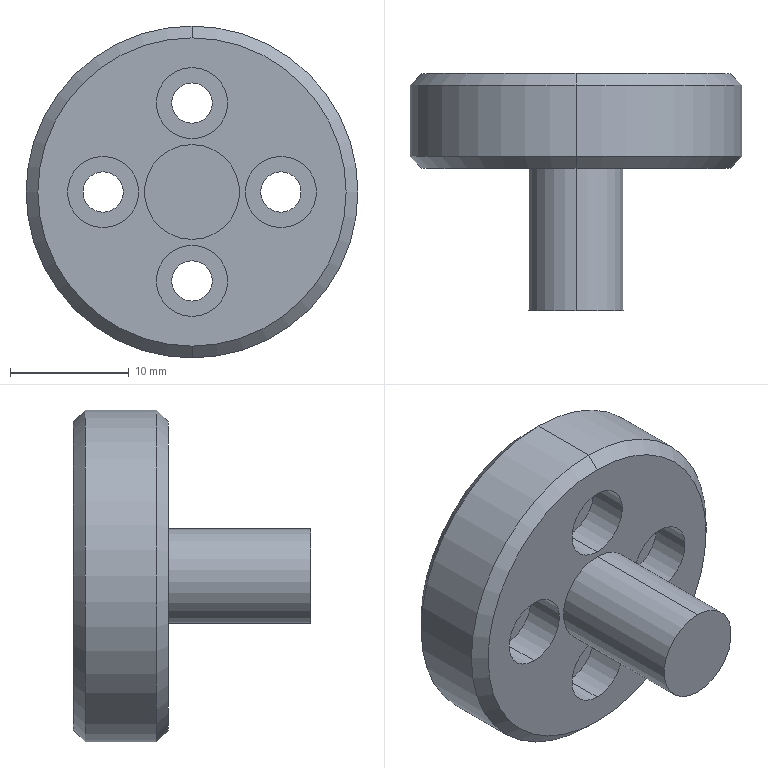Component | SolidWorks | H2020022-0438-1-1 | 1 solid | 34 faces | box 28 x 20 x 28 mm | volume 4336 mm3 | cylinder 22 | plane 8 | cone 4 | commonest cylinder face diameters 6 x8 3.4 x8 8 x2 20 x2 28 x2 | material 45#Steel
build123d program:
from build123d import *

# Parameters (mm, degrees)
SKETCH1_R                                       = 14
BOSS_EXTRUDE1_DEPTH                             = 8
SKETCH2_R                                       = 10
CUT_EXTRUDE1_DEPTH                              = 2
M3_HEX_SOCKET_HEAD_CAP_SCREW_CBORE1_D           = 3.4
M3_HEX_SOCKET_HEAD_CAP_SCREW_CBORE1_CBORE_D     = 6
M3_HEX_SOCKET_HEAD_CAP_SCREW_CBORE1_CBORE_DEPTH = 3.4
SKETCH5_R                                       = 4
BOSS_EXTRUDE2_DEPTH                             = 12
CHAMFER1_SIZE                                   = 1


with BuildPart() as part:
    # Sketch1 → Boss-Extrude1 (new body)
    with BuildSketch(Plane(origin=(0, 0, 0), x_dir=(1, 0, 0), z_dir=(0, 1, 0))):
        with Locations(Location((0, 0, 0), (0, 0, 270))):
            Circle(SKETCH1_R)
    extrude(amount=BOSS_EXTRUDE1_DEPTH)

    # Sketch2 → Cut-Extrude1 (cut)
    with BuildSketch(Plane(origin=(0, 8, 0), x_dir=(1, 0, 0), z_dir=(0, 1, 0))):
        with Locations(Location((0, 0, 0), (0, 0, 270))):
            Circle(SKETCH2_R)
    extrude(amount=-CUT_EXTRUDE1_DEPTH, mode=Mode.SUBTRACT)

    # M3 Hex Socket Head Cap Screw CBORE1 (through all)
    with Locations(Plane(origin=(0, 0, 0), x_dir=(-1, 0, 0), z_dir=(0, -1, 0))):
        with Locations((0, 7.5), (0, -7.5), (-7.5, 0), (7.5, 0)):
            CounterBoreHole(M3_HEX_SOCKET_HEAD_CAP_SCREW_CBORE1_D / 2, M3_HEX_SOCKET_HEAD_CAP_SCREW_CBORE1_CBORE_D / 2, M3_HEX_SOCKET_HEAD_CAP_SCREW_CBORE1_CBORE_DEPTH)

    # Sketch5 → Boss-Extrude2 (add)
    with BuildSketch(Plane.XZ):
        with Locations(Location((0, 0, 0), (0, 0, 90))):
            Circle(SKETCH5_R)
    extrude(amount=BOSS_EXTRUDE2_DEPTH)

    # Chamfer1
    chamfer1_edges = [part.edges().sort_by_distance(p)[0] for p in [
        (0, 0, -14),
        (0, 8, -14),
    ]]
    chamfer(chamfer1_edges, length=CHAMFER1_SIZE)


solid = part.part

# Placed as in the assembly
solid = solid.moved(Location((-30.964, 93.813, 280.197), (0, 0, 0)))
STEP:
#1=CARTESIAN_POINT('',(-1.219,4.008,11.543));
#2=VERTEX_POINT('',#1);
#3=CARTESIAN_POINT('',(-1.219,4.008,10.52));
#4=VERTEX_POINT('',#3);
#5=CARTESIAN_POINT('',(-1.219,4.008,11.031));
#6=DIRECTION('',(0.,1.,0.));
#7=DIRECTION('',(0.,0.,1.));
#8=AXIS2_PLACEMENT_3D('',#5,#6,#7);
#9=CIRCLE('',#8,0.5118);
#10=EDGE_CURVE('',#2,#4,#9,.T.);
#11=ORIENTED_EDGE('',*,*,#10,.F.);
#12=CARTESIAN_POINT('',(-1.219,3.969,11.583));
#13=VERTEX_POINT('',#12);
#14=CARTESIAN_POINT('',(-1.219,4.008,11.543));
#15=DIRECTION('',(0.,-0.7071,0.7071));
#16=VECTOR('',#15,39.37);
#17=LINE('',#14,#16);
#18=EDGE_CURVE('',#2,#13,#17,.T.);
#19=ORIENTED_EDGE('',*,*,#18,.T.);
#20=CARTESIAN_POINT('',(-1.219,3.969,10.48));
#21=VERTEX_POINT('',#20);
#22=CARTESIAN_POINT('',(-1.219,3.969,11.031));
#23=DIRECTION('',(0.,-1.,0.));
#24=DIRECTION('',(0.,0.,1.));
#25=AXIS2_PLACEMENT_3D('',#22,#23,#24);
#26=CIRCLE('',#25,0.5512);
#27=EDGE_CURVE('',#21,#13,#26,.T.);
#28=ORIENTED_EDGE('',*,*,#27,.F.);
#29=CARTESIAN_POINT('',(-1.219,4.008,10.52));
#30=DIRECTION('',(0.,-0.7071,-0.7071));
#31=VECTOR('',#30,39.37);
#32=LINE('',#29,#31);
#33=EDGE_CURVE('',#4,#21,#32,.T.);
#34=ORIENTED_EDGE('',*,*,#33,.F.);
#35=EDGE_LOOP('',(#11,#19,#28,#34));
#36=FACE_OUTER_BOUND('',#35,.T.);
#37=CARTESIAN_POINT('',(-1.219,4.008,11.031));
#38=DIRECTION('',(0.,-1.,0.));
#39=DIRECTION('',(0.,0.,-1.));
#40=AXIS2_PLACEMENT_3D('',#37,#38,#39);
#41=CONICAL_SURFACE('',#40,0.5118,0.7854);
#42=ADVANCED_FACE('',(#36),#41,.T.);
#43=CARTESIAN_POINT('',(-1.219,3.693,10.52));
#44=VERTEX_POINT('',#43);
#45=CARTESIAN_POINT('',(-1.219,3.693,11.543));
#46=VERTEX_POINT('',#45);
#47=CARTESIAN_POINT('',(-1.219,3.693,11.031));
#48=DIRECTION('',(0.,-1.,0.));
#49=DIRECTION('',(0.,0.,1.));
#50=AXIS2_PLACEMENT_3D('',#47,#48,#49);
#51=CIRCLE('',#50,0.5118);
#52=EDGE_CURVE('',#44,#46,#51,.T.);
#53=ORIENTED_EDGE('',*,*,#52,.F.);
#54=CARTESIAN_POINT('',(-1.219,3.733,10.48));
#55=VERTEX_POINT('',#54);
#56=CARTESIAN_POINT('',(-1.219,3.733,10.48));
#57=DIRECTION('',(0.,0.7071,-0.7071));
#58=VECTOR('',#57,39.37);
#59=LINE('',#56,#58);
#60=EDGE_CURVE('',#44,#55,#59,.T.);
#61=ORIENTED_EDGE('',*,*,#60,.T.);
#62=CARTESIAN_POINT('',(-1.219,3.733,11.583));
#63=VERTEX_POINT('',#62);
#64=CARTESIAN_POINT('',(-1.219,3.733,11.031));
#65=DIRECTION('',(0.,1.,0.));
#66=DIRECTION('',(0.,0.,1.));
#67=AXIS2_PLACEMENT_3D('',#64,#65,#66);
#68=CIRCLE('',#67,0.5512);
#69=EDGE_CURVE('',#63,#55,#68,.T.);
#70=ORIENTED_EDGE('',*,*,#69,.F.);
#71=CARTESIAN_POINT('',(-1.219,3.733,11.583));
#72=DIRECTION('',(0.,0.7071,0.7071));
#73=VECTOR('',#72,39.37);
#74=LINE('',#71,#73);
#75=EDGE_CURVE('',#46,#63,#74,.T.);
#76=ORIENTED_EDGE('',*,*,#75,.F.);
#77=EDGE_LOOP('',(#53,#61,#70,#76));
#78=FACE_OUTER_BOUND('',#77,.T.);
#79=CARTESIAN_POINT('',(-1.219,3.733,11.031));
#80=DIRECTION('',(0.,1.,0.));
#81=DIRECTION('',(0.,0.,1.));
#82=AXIS2_PLACEMENT_3D('',#79,#80,#81);
#83=CONICAL_SURFACE('',#82,0.5512,0.7854);
#84=ADVANCED_FACE('',(#78),#83,.T.);
#85=CARTESIAN_POINT('',(-1.219,3.221,10.874));
#86=VERTEX_POINT('',#85);
#87=CARTESIAN_POINT('',(-1.219,3.221,11.189));
#88=VERTEX_POINT('',#87);
#89=CARTESIAN_POINT('',(-1.219,3.221,11.031));
#90=DIRECTION('',(0.,-1.,0.));
#91=DIRECTION('',(0.,0.,-1.));
#92=AXIS2_PLACEMENT_3D('',#89,#90,#91);
#93=CIRCLE('',#92,0.1575);
#94=EDGE_CURVE('',#86,#88,#93,.T.);
#95=ORIENTED_EDGE('',*,*,#94,.F.);
#96=CARTESIAN_POINT('',(-1.219,3.693,10.874));
#97=VERTEX_POINT('',#96);
#98=CARTESIAN_POINT('',(-1.219,3.221,10.874));
#99=DIRECTION('',(0.,1.,0.));
#100=VECTOR('',#99,39.37);
#101=LINE('',#98,#100);
#102=EDGE_CURVE('',#86,#97,#101,.T.);
#103=ORIENTED_EDGE('',*,*,#102,.T.);
#104=CARTESIAN_POINT('',(-1.219,3.693,11.189));
#105=VERTEX_POINT('',#104);
#106=CARTESIAN_POINT('',(-1.219,3.693,11.031));
#107=DIRECTION('',(0.,-1.,0.));
#108=DIRECTION('',(0.,0.,1.));
#109=AXIS2_PLACEMENT_3D('',#106,#107,#108);
#110=CIRCLE('',#109,0.1575);
#111=EDGE_CURVE('',#97,#105,#110,.T.);
#112=ORIENTED_EDGE('',*,*,#111,.T.);
#113=CARTESIAN_POINT('',(-1.219,3.221,11.189));
#114=DIRECTION('',(0.,1.,0.));
#115=VECTOR('',#114,39.37);
#116=LINE('',#113,#115);
#117=EDGE_CURVE('',#88,#105,#116,.T.);
#118=ORIENTED_EDGE('',*,*,#117,.F.);
#119=EDGE_LOOP('',(#95,#103,#112,#118));
#120=FACE_OUTER_BOUND('',#119,.T.);
#121=CARTESIAN_POINT('',(-1.219,3.221,11.031));
#122=DIRECTION('',(0.,1.,0.));
#123=DIRECTION('',(0.,0.,1.));
#124=AXIS2_PLACEMENT_3D('',#121,#122,#123);
#125=CYLINDRICAL_SURFACE('',#124,0.1575);
#126=ADVANCED_FACE('',(#120),#125,.T.);
#127=CARTESIAN_POINT('',(-1.219,3.827,10.854));
#128=VERTEX_POINT('',#127);
#129=CARTESIAN_POINT('',(-1.219,3.827,10.618));
#130=VERTEX_POINT('',#129);
#131=CARTESIAN_POINT('',(-1.219,3.827,10.736));
#132=DIRECTION('',(0.,-1.,0.));
#133=DIRECTION('',(0.,0.,-1.));
#134=AXIS2_PLACEMENT_3D('',#131,#132,#133);
#135=CIRCLE('',#134,0.1181);
#136=EDGE_CURVE('',#128,#130,#135,.T.);
#137=ORIENTED_EDGE('',*,*,#136,.F.);
#138=CARTESIAN_POINT('',(-1.219,3.693,10.854));
#139=VERTEX_POINT('',#138);
#140=CARTESIAN_POINT('',(-1.219,3.693,10.854));
#141=DIRECTION('',(0.,-1.,0.));
#142=VECTOR('',#141,39.37);
#143=LINE('',#140,#142);
#144=EDGE_CURVE('',#128,#139,#143,.T.);
#145=ORIENTED_EDGE('',*,*,#144,.T.);
#146=CARTESIAN_POINT('',(-1.219,3.693,10.618));
#147=VERTEX_POINT('',#146);
#148=CARTESIAN_POINT('',(-1.219,3.693,10.736));
#149=DIRECTION('',(0.,-1.,0.));
#150=DIRECTION('',(0.,0.,-1.));
#151=AXIS2_PLACEMENT_3D('',#148,#149,#150);
#152=CIRCLE('',#151,0.1181);
#153=EDGE_CURVE('',#139,#147,#152,.T.);
#154=ORIENTED_EDGE('',*,*,#153,.T.);
#155=CARTESIAN_POINT('',(-1.219,3.693,10.618));
#156=DIRECTION('',(0.,-1.,0.));
#157=VECTOR('',#156,39.37);
#158=LINE('',#155,#157);
#159=EDGE_CURVE('',#130,#147,#158,.T.);
#160=ORIENTED_EDGE('',*,*,#159,.F.);
#161=EDGE_LOOP('',(#137,#145,#154,#160));
#162=FACE_OUTER_BOUND('',#161,.T.);
#163=CARTESIAN_POINT('',(-1.219,3.693,10.736));
#164=DIRECTION('',(0.,-1.,0.));
#165=DIRECTION('',(0.,0.,-1.));
#166=AXIS2_PLACEMENT_3D('',#163,#164,#165);
#167=CYLINDRICAL_SURFACE('',#166,0.1181);
#168=ADVANCED_FACE('',(#162),#167,.F.);
#169=CARTESIAN_POINT('',(-1.219,3.93,10.669));
#170=VERTEX_POINT('',#169);
#171=CARTESIAN_POINT('',(-1.219,3.93,10.803));
#172=VERTEX_POINT('',#171);
#173=CARTESIAN_POINT('',(-1.219,3.93,10.736));
#174=DIRECTION('',(0.,1.,0.));
#175=DIRECTION('',(0.,0.,1.));
#176=AXIS2_PLACEMENT_3D('',#173,#174,#175);
#177=CIRCLE('',#176,0.06693);
#178=EDGE_CURVE('',#170,#172,#177,.T.);
#179=ORIENTED_EDGE('',*,*,#178,.T.);
#180=CARTESIAN_POINT('',(-1.219,3.827,10.803));
#181=VERTEX_POINT('',#180);
#182=CARTESIAN_POINT('',(-1.219,3.693,10.803));
#183=DIRECTION('',(0.,-1.,0.));
#184=VECTOR('',#183,39.37);
#185=LINE('',#182,#184);
#186=EDGE_CURVE('',#172,#181,#185,.T.);
#187=ORIENTED_EDGE('',*,*,#186,.T.);
#188=CARTESIAN_POINT('',(-1.219,3.827,10.669));
#189=VERTEX_POINT('',#188);
#190=CARTESIAN_POINT('',(-1.219,3.827,10.736));
#191=DIRECTION('',(0.,-1.,0.));
#192=DIRECTION('',(0.,0.,-1.));
#193=AXIS2_PLACEMENT_3D('',#190,#191,#192);
#194=CIRCLE('',#193,0.06693);
#195=EDGE_CURVE('',#181,#189,#194,.T.);
#196=ORIENTED_EDGE('',*,*,#195,.T.);
#197=CARTESIAN_POINT('',(-1.219,3.693,10.669));
#198=DIRECTION('',(0.,-1.,0.));
#199=VECTOR('',#198,39.37);
#200=LINE('',#197,#199);
#201=EDGE_CURVE('',#170,#189,#200,.T.);
#202=ORIENTED_EDGE('',*,*,#201,.F.);
#203=EDGE_LOOP('',(#179,#187,#196,#202));
#204=FACE_OUTER_BOUND('',#203,.T.);
#205=CARTESIAN_POINT('',(-1.219,3.693,10.736));
#206=DIRECTION('',(0.,-1.,0.));
#207=DIRECTION('',(0.,0.,-1.));
#208=AXIS2_PLACEMENT_3D('',#205,#206,#207);
#209=CYLINDRICAL_SURFACE('',#208,0.06693);
#210=ADVANCED_FACE('',(#204),#209,.F.);
#211=CARTESIAN_POINT('',(-1.219,3.827,11.445));
#212=VERTEX_POINT('',#211);
#213=CARTESIAN_POINT('',(-1.219,3.827,11.209));
#214=VERTEX_POINT('',#213);
#215=CARTESIAN_POINT('',(-1.219,3.827,11.327));
#216=DIRECTION('',(0.,-1.,0.));
#217=DIRECTION('',(0.,0.,-1.));
#218=AXIS2_PLACEMENT_3D('',#215,#216,#217);
#219=CIRCLE('',#218,0.1181);
#220=EDGE_CURVE('',#212,#214,#219,.T.);
#221=ORIENTED_EDGE('',*,*,#220,.F.);
#222=CARTESIAN_POINT('',(-1.219,3.693,11.445));
#223=VERTEX_POINT('',#222);
#224=CARTESIAN_POINT('',(-1.219,3.693,11.445));
#225=DIRECTION('',(0.,-1.,0.));
#226=VECTOR('',#225,39.37);
#227=LINE('',#224,#226);
#228=EDGE_CURVE('',#212,#223,#227,.T.);
#229=ORIENTED_EDGE('',*,*,#228,.T.);
#230=CARTESIAN_POINT('',(-1.219,3.693,11.209));
#231=VERTEX_POINT('',#230);
#232=CARTESIAN_POINT('',(-1.219,3.693,11.327));
#233=DIRECTION('',(0.,-1.,0.));
#234=DIRECTION('',(0.,0.,-1.));
#235=AXIS2_PLACEMENT_3D('',#232,#233,#234);
#236=CIRCLE('',#235,0.1181);
#237=EDGE_CURVE('',#223,#231,#236,.T.);
#238=ORIENTED_EDGE('',*,*,#237,.T.);
#239=CARTESIAN_POINT('',(-1.219,3.693,11.209));
#240=DIRECTION('',(0.,-1.,0.));
#241=VECTOR('',#240,39.37);
#242=LINE('',#239,#241);
#243=EDGE_CURVE('',#214,#231,#242,.T.);
#244=ORIENTED_EDGE('',*,*,#243,.F.);
#245=EDGE_LOOP('',(#221,#229,#238,#244));
#246=FACE_OUTER_BOUND('',#245,.T.);
#247=CARTESIAN_POINT('',(-1.219,3.693,11.327));
#248=DIRECTION('',(0.,-1.,0.));
#249=DIRECTION('',(0.,0.,-1.));
#250=AXIS2_PLACEMENT_3D('',#247,#248,#249);
#251=CYLINDRICAL_SURFACE('',#250,0.1181);
#252=ADVANCED_FACE('',(#246),#251,.F.);
#253=CARTESIAN_POINT('',(-1.219,3.93,11.26));
#254=VERTEX_POINT('',#253);
#255=CARTESIAN_POINT('',(-1.219,3.93,11.394));
#256=VERTEX_POINT('',#255);
#257=CARTESIAN_POINT('',(-1.219,3.93,11.327));
#258=DIRECTION('',(0.,1.,0.));
#259=DIRECTION('',(0.,0.,1.));
#260=AXIS2_PLACEMENT_3D('',#257,#258,#259);
#261=CIRCLE('',#260,0.06693);
#262=EDGE_CURVE('',#254,#256,#261,.T.);
#263=ORIENTED_EDGE('',*,*,#262,.T.);
#264=CARTESIAN_POINT('',(-1.219,3.827,11.394));
#265=VERTEX_POINT('',#264);
#266=CARTESIAN_POINT('',(-1.219,3.693,11.394));
#267=DIRECTION('',(0.,-1.,0.));
#268=VECTOR('',#267,39.37);
#269=LINE('',#266,#268);
#270=EDGE_CURVE('',#256,#265,#269,.T.);
#271=ORIENTED_EDGE('',*,*,#270,.T.);
#272=CARTESIAN_POINT('',(-1.219,3.827,11.26));
#273=VERTEX_POINT('',#272);
#274=CARTESIAN_POINT('',(-1.219,3.827,11.327));
#275=DIRECTION('',(0.,-1.,0.));
#276=DIRECTION('',(0.,0.,-1.));
#277=AXIS2_PLACEMENT_3D('',#274,#275,#276);
#278=CIRCLE('',#277,0.06693);
#279=EDGE_CURVE('',#265,#273,#278,.T.);
#280=ORIENTED_EDGE('',*,*,#279,.T.);
#281=CARTESIAN_POINT('',(-1.219,3.693,11.26));
#282=DIRECTION('',(0.,-1.,0.));
#283=VECTOR('',#282,39.37);
#284=LINE('',#281,#283);
#285=EDGE_CURVE('',#254,#273,#284,.T.);
#286=ORIENTED_EDGE('',*,*,#285,.F.);
#287=EDGE_LOOP('',(#263,#271,#280,#286));
#288=FACE_OUTER_BOUND('',#287,.T.);
#289=CARTESIAN_POINT('',(-1.219,3.693,11.327));
#290=DIRECTION('',(0.,-1.,0.));
#291=DIRECTION('',(0.,0.,-1.));
#292=AXIS2_PLACEMENT_3D('',#289,#290,#291);
#293=CYLINDRICAL_SURFACE('',#292,0.06693);
#294=ADVANCED_FACE('',(#288),#293,.F.);
#295=CARTESIAN_POINT('',(-0.9238,3.827,11.149));
#296=VERTEX_POINT('',#295);
#297=CARTESIAN_POINT('',(-0.9238,3.827,10.913));
#298=VERTEX_POINT('',#297);
#299=CARTESIAN_POINT('',(-0.9238,3.827,11.031));
#300=DIRECTION('',(0.,-1.,0.));
#301=DIRECTION('',(0.,0.,-1.));
#302=AXIS2_PLACEMENT_3D('',#299,#300,#301);
#303=CIRCLE('',#302,0.1181);
#304=EDGE_CURVE('',#296,#298,#303,.T.);
#305=ORIENTED_EDGE('',*,*,#304,.F.);
#306=CARTESIAN_POINT('',(-0.9238,3.693,11.149));
#307=VERTEX_POINT('',#306);
#308=CARTESIAN_POINT('',(-0.9238,3.693,11.149));
#309=DIRECTION('',(0.,-1.,0.));
#310=VECTOR('',#309,39.37);
#311=LINE('',#308,#310);
#312=EDGE_CURVE('',#296,#307,#311,.T.);
#313=ORIENTED_EDGE('',*,*,#312,.T.);
#314=CARTESIAN_POINT('',(-0.9238,3.693,10.913));
#315=VERTEX_POINT('',#314);
#316=CARTESIAN_POINT('',(-0.9238,3.693,11.031));
#317=DIRECTION('',(0.,-1.,0.));
#318=DIRECTION('',(0.,0.,-1.));
#319=AXIS2_PLACEMENT_3D('',#316,#317,#318);
#320=CIRCLE('',#319,0.1181);
#321=EDGE_CURVE('',#307,#315,#320,.T.);
#322=ORIENTED_EDGE('',*,*,#321,.T.);
#323=CARTESIAN_POINT('',(-0.9238,3.693,10.913));
#324=DIRECTION('',(0.,-1.,0.));
#325=VECTOR('',#324,39.37);
#326=LINE('',#323,#325);
#327=EDGE_CURVE('',#298,#315,#326,.T.);
#328=ORIENTED_EDGE('',*,*,#327,.F.);
#329=EDGE_LOOP('',(#305,#313,#322,#328));
#330=FACE_OUTER_BOUND('',#329,.T.);
#331=CARTESIAN_POINT('',(-0.9238,3.693,11.031));
#332=DIRECTION('',(0.,-1.,0.));
#333=DIRECTION('',(0.,0.,-1.));
#334=AXIS2_PLACEMENT_3D('',#331,#332,#333);
#335=CYLINDRICAL_SURFACE('',#334,0.1181);
#336=ADVANCED_FACE('',(#330),#335,.F.);
#337=CARTESIAN_POINT('',(-0.9238,3.93,10.964));
#338=VERTEX_POINT('',#337);
#339=CARTESIAN_POINT('',(-0.9238,3.93,11.098));
#340=VERTEX_POINT('',#339);
#341=CARTESIAN_POINT('',(-0.9238,3.93,11.031));
#342=DIRECTION('',(0.,1.,0.));
#343=DIRECTION('',(0.,0.,1.));
#344=AXIS2_PLACEMENT_3D('',#341,#342,#343);
#345=CIRCLE('',#344,0.06693);
#346=EDGE_CURVE('',#338,#340,#345,.T.);
#347=ORIENTED_EDGE('',*,*,#346,.T.);
#348=CARTESIAN_POINT('',(-0.9238,3.827,11.098));
#349=VERTEX_POINT('',#348);
#350=CARTESIAN_POINT('',(-0.9238,3.693,11.098));
#351=DIRECTION('',(0.,-1.,0.));
#352=VECTOR('',#351,39.37);
#353=LINE('',#350,#352);
#354=EDGE_CURVE('',#340,#349,#353,.T.);
#355=ORIENTED_EDGE('',*,*,#354,.T.);
#356=CARTESIAN_POINT('',(-0.9238,3.827,10.964));
#357=VERTEX_POINT('',#356);
#358=CARTESIAN_POINT('',(-0.9238,3.827,11.031));
#359=DIRECTION('',(0.,-1.,0.));
#360=DIRECTION('',(0.,0.,-1.));
#361=AXIS2_PLACEMENT_3D('',#358,#359,#360);
#362=CIRCLE('',#361,0.06693);
#363=EDGE_CURVE('',#349,#357,#362,.T.);
#364=ORIENTED_EDGE('',*,*,#363,.T.);
#365=CARTESIAN_POINT('',(-0.9238,3.693,10.964));
#366=DIRECTION('',(0.,-1.,0.));
#367=VECTOR('',#366,39.37);
#368=LINE('',#365,#367);
#369=EDGE_CURVE('',#338,#357,#368,.T.);
#370=ORIENTED_EDGE('',*,*,#369,.F.);
#371=EDGE_LOOP('',(#347,#355,#364,#370));
#372=FACE_OUTER_BOUND('',#371,.T.);
#373=CARTESIAN_POINT('',(-0.9238,3.693,11.031));
#374=DIRECTION('',(0.,-1.,0.));
#375=DIRECTION('',(0.,0.,-1.));
#376=AXIS2_PLACEMENT_3D('',#373,#374,#375);
#377=CYLINDRICAL_SURFACE('',#376,0.06693);
#378=ADVANCED_FACE('',(#372),#377,.F.);
#379=CARTESIAN_POINT('',(-1.514,3.827,11.149));
#380=VERTEX_POINT('',#379);
#381=CARTESIAN_POINT('',(-1.514,3.827,10.913));
#382=VERTEX_POINT('',#381);
#383=CARTESIAN_POINT('',(-1.514,3.827,11.031));
#384=DIRECTION('',(0.,-1.,0.));
#385=DIRECTION('',(0.,0.,-1.));
#386=AXIS2_PLACEMENT_3D('',#383,#384,#385);
#387=CIRCLE('',#386,0.1181);
#388=EDGE_CURVE('',#380,#382,#387,.T.);
#389=ORIENTED_EDGE('',*,*,#388,.F.);
#390=CARTESIAN_POINT('',(-1.514,3.693,11.149));
#391=VERTEX_POINT('',#390);
#392=CARTESIAN_POINT('',(-1.514,3.693,11.149));
#393=DIRECTION('',(0.,-1.,0.));
#394=VECTOR('',#393,39.37);
#395=LINE('',#392,#394);
#396=EDGE_CURVE('',#380,#391,#395,.T.);
#397=ORIENTED_EDGE('',*,*,#396,.T.);
#398=CARTESIAN_POINT('',(-1.514,3.693,10.913));
#399=VERTEX_POINT('',#398);
#400=CARTESIAN_POINT('',(-1.514,3.693,11.031));
#401=DIRECTION('',(0.,-1.,0.));
#402=DIRECTION('',(0.,0.,-1.));
#403=AXIS2_PLACEMENT_3D('',#400,#401,#402);
#404=CIRCLE('',#403,0.1181);
#405=EDGE_CURVE('',#391,#399,#404,.T.);
#406=ORIENTED_EDGE('',*,*,#405,.T.);
#407=CARTESIAN_POINT('',(-1.514,3.693,10.913));
#408=DIRECTION('',(0.,-1.,0.));
#409=VECTOR('',#408,39.37);
#410=LINE('',#407,#409);
#411=EDGE_CURVE('',#382,#399,#410,.T.);
#412=ORIENTED_EDGE('',*,*,#411,.F.);
#413=EDGE_LOOP('',(#389,#397,#406,#412));
#414=FACE_OUTER_BOUND('',#413,.T.);
#415=CARTESIAN_POINT('',(-1.514,3.693,11.031));
#416=DIRECTION('',(0.,-1.,0.));
#417=DIRECTION('',(0.,0.,-1.));
#418=AXIS2_PLACEMENT_3D('',#415,#416,#417);
#419=CYLINDRICAL_SURFACE('',#418,0.1181);
#420=ADVANCED_FACE('',(#414),#419,.F.);
#421=CARTESIAN_POINT('',(-1.514,3.93,10.964));
#422=VERTEX_POINT('',#421);
#423=CARTESIAN_POINT('',(-1.514,3.93,11.098));
#424=VERTEX_POINT('',#423);
#425=CARTESIAN_POINT('',(-1.514,3.93,11.031));
#426=DIRECTION('',(0.,1.,0.));
#427=DIRECTION('',(0.,0.,1.));
#428=AXIS2_PLACEMENT_3D('',#425,#426,#427);
#429=CIRCLE('',#428,0.06693);
#430=EDGE_CURVE('',#422,#424,#429,.T.);
#431=ORIENTED_EDGE('',*,*,#430,.T.);
#432=CARTESIAN_POINT('',(-1.514,3.827,11.098));
#433=VERTEX_POINT('',#432);
#434=CARTESIAN_POINT('',(-1.514,3.693,11.098));
#435=DIRECTION('',(0.,-1.,0.));
#436=VECTOR('',#435,39.37);
#437=LINE('',#434,#436);
#438=EDGE_CURVE('',#424,#433,#437,.T.);
#439=ORIENTED_EDGE('',*,*,#438,.T.);
#440=CARTESIAN_POINT('',(-1.514,3.827,10.964));
#441=VERTEX_POINT('',#440);
#442=CARTESIAN_POINT('',(-1.514,3.827,11.031));
#443=DIRECTION('',(0.,-1.,0.));
#444=DIRECTION('',(0.,0.,-1.));
#445=AXIS2_PLACEMENT_3D('',#442,#443,#444);
#446=CIRCLE('',#445,0.06693);
#447=EDGE_CURVE('',#433,#441,#446,.T.);
#448=ORIENTED_EDGE('',*,*,#447,.T.);
#449=CARTESIAN_POINT('',(-1.514,3.693,10.964));
#450=DIRECTION('',(0.,-1.,0.));
#451=VECTOR('',#450,39.37);
#452=LINE('',#449,#451);
#453=EDGE_CURVE('',#422,#441,#452,.T.);
#454=ORIENTED_EDGE('',*,*,#453,.F.);
#455=EDGE_LOOP('',(#431,#439,#448,#454));
#456=FACE_OUTER_BOUND('',#455,.T.);
#457=CARTESIAN_POINT('',(-1.514,3.693,11.031));
#458=DIRECTION('',(0.,-1.,0.));
#459=DIRECTION('',(0.,0.,-1.));
#460=AXIS2_PLACEMENT_3D('',#457,#458,#459);
#461=CYLINDRICAL_SURFACE('',#460,0.06693);
#462=ADVANCED_FACE('',(#456),#461,.F.);
#463=CARTESIAN_POINT('',(-1.219,3.93,10.638));
#464=VERTEX_POINT('',#463);
#465=CARTESIAN_POINT('',(-1.219,3.93,11.425));
#466=VERTEX_POINT('',#465);
#467=CARTESIAN_POINT('',(-1.219,3.93,11.031));
#468=DIRECTION('',(0.,1.,0.));
#469=DIRECTION('',(0.,0.,1.));
#470=AXIS2_PLACEMENT_3D('',#467,#468,#469);
#471=CIRCLE('',#470,0.3937);
#472=EDGE_CURVE('',#464,#466,#471,.T.);
#473=ORIENTED_EDGE('',*,*,#472,.F.);
#474=CARTESIAN_POINT('',(-1.219,4.008,10.638));
#475=VERTEX_POINT('',#474);
#476=CARTESIAN_POINT('',(-1.219,3.93,10.638));
#477=DIRECTION('',(0.,1.,0.));
#478=VECTOR('',#477,39.37);
#479=LINE('',#476,#478);
#480=EDGE_CURVE('',#464,#475,#479,.T.);
#481=ORIENTED_EDGE('',*,*,#480,.T.);
#482=CARTESIAN_POINT('',(-1.219,4.008,11.425));
#483=VERTEX_POINT('',#482);
#484=CARTESIAN_POINT('',(-1.219,4.008,11.031));
#485=DIRECTION('',(0.,1.,0.));
#486=DIRECTION('',(0.,0.,1.));
#487=AXIS2_PLACEMENT_3D('',#484,#485,#486);
#488=CIRCLE('',#487,0.3937);
#489=EDGE_CURVE('',#475,#483,#488,.T.);
#490=ORIENTED_EDGE('',*,*,#489,.T.);
#491=CARTESIAN_POINT('',(-1.219,3.93,11.425));
#492=DIRECTION('',(0.,1.,0.));
#493=VECTOR('',#492,39.37);
#494=LINE('',#491,#493);
#495=EDGE_CURVE('',#466,#483,#494,.T.);
#496=ORIENTED_EDGE('',*,*,#495,.F.);
#497=EDGE_LOOP('',(#473,#481,#490,#496));
#498=FACE_OUTER_BOUND('',#497,.T.);
#499=CARTESIAN_POINT('',(-1.219,3.93,11.031));
#500=DIRECTION('',(0.,1.,0.));
#501=DIRECTION('',(0.,0.,1.));
#502=AXIS2_PLACEMENT_3D('',#499,#500,#501);
#503=CYLINDRICAL_SURFACE('',#502,0.3937);
#504=ADVANCED_FACE('',(#498),#503,.F.);
#505=ORIENTED_EDGE('',*,*,#27,.T.);
#506=CARTESIAN_POINT('',(-1.219,4.008,11.583));
#507=DIRECTION('',(0.,-1.,0.));
#508=VECTOR('',#507,39.37);
#509=LINE('',#506,#508);
#510=EDGE_CURVE('',#13,#63,#509,.T.);
#511=ORIENTED_EDGE('',*,*,#510,.T.);
#512=ORIENTED_EDGE('',*,*,#69,.T.);
#513=CARTESIAN_POINT('',(-1.219,4.008,10.48));
#514=DIRECTION('',(0.,-1.,0.));
#515=VECTOR('',#514,39.37);
#516=LINE('',#513,#515);
#517=EDGE_CURVE('',#21,#55,#516,.T.);
#518=ORIENTED_EDGE('',*,*,#517,.F.);
#519=EDGE_LOOP('',(#505,#511,#512,#518));
#520=FACE_OUTER_BOUND('',#519,.T.);
#521=CARTESIAN_POINT('',(-1.219,4.008,11.031));
#522=DIRECTION('',(0.,-1.,0.));
#523=DIRECTION('',(0.,0.,-1.));
#524=AXIS2_PLACEMENT_3D('',#521,#522,#523);
#525=CYLINDRICAL_SURFACE('',#524,0.5512);
#526=ADVANCED_FACE('',(#520),#525,.T.);
#527=ORIENTED_EDGE('',*,*,#510,.F.);
#528=CARTESIAN_POINT('',(-1.219,3.969,11.031));
#529=DIRECTION('',(0.,-1.,0.));
#530=DIRECTION('',(0.,0.,1.));
#531=AXIS2_PLACEMENT_3D('',#528,#529,#530);
#532=CIRCLE('',#531,0.5512);
#533=EDGE_CURVE('',#13,#21,#532,.T.);
#534=ORIENTED_EDGE('',*,*,#533,.T.);
#535=ORIENTED_EDGE('',*,*,#517,.T.);
#536=CARTESIAN_POINT('',(-1.219,3.733,11.031));
#537=DIRECTION('',(0.,1.,0.));
#538=DIRECTION('',(0.,0.,1.));
#539=AXIS2_PLACEMENT_3D('',#536,#537,#538);
#540=CIRCLE('',#539,0.5512);
#541=EDGE_CURVE('',#55,#63,#540,.T.);
#542=ORIENTED_EDGE('',*,*,#541,.T.);
#543=EDGE_LOOP('',(#527,#534,#535,#542));
#544=FACE_OUTER_BOUND('',#543,.T.);
#545=CARTESIAN_POINT('',(-1.219,4.008,11.031));
#546=DIRECTION('',(0.,-1.,0.));
#547=DIRECTION('',(0.,0.,-1.));
#548=AXIS2_PLACEMENT_3D('',#545,#546,#547);
#549=CYLINDRICAL_SURFACE('',#548,0.5512);
#550=ADVANCED_FACE('',(#544),#549,.T.);
#551=CARTESIAN_POINT('',(-1.219,4.008,11.031));
#552=DIRECTION('',(0.,1.,0.));
#553=DIRECTION('',(0.,0.,1.));
#554=AXIS2_PLACEMENT_3D('',#551,#552,#553);
#555=CIRCLE('',#554,0.5118);
#556=EDGE_CURVE('',#4,#2,#555,.T.);
#557=ORIENTED_EDGE('',*,*,#556,.T.);
#558=ORIENTED_EDGE('',*,*,#10,.T.);
#559=EDGE_LOOP('',(#557,#558));
#560=FACE_OUTER_BOUND('',#559,.T.);
#561=CARTESIAN_POINT('',(-1.219,4.008,11.031));
#562=DIRECTION('',(0.,1.,0.));
#563=DIRECTION('',(0.,0.,1.));
#564=AXIS2_PLACEMENT_3D('',#561,#562,#563);
#565=CIRCLE('',#564,0.3937);
#566=EDGE_CURVE('',#483,#475,#565,.T.);
#567=ORIENTED_EDGE('',*,*,#566,.F.);
#568=ORIENTED_EDGE('',*,*,#489,.F.);
#569=EDGE_LOOP('',(#567,#568));
#570=FACE_BOUND('',#569,.T.);
#571=CARTESIAN_POINT('',(-1.219,4.008,11.031));
#572=DIRECTION('',(0.,1.,0.));
#573=DIRECTION('',(0.,0.,1.));
#574=AXIS2_PLACEMENT_3D('',#571,#572,#573);
#575=PLANE('',#574);
#576=ADVANCED_FACE('',(#560,#570),#575,.T.);
#577=CARTESIAN_POINT('',(-1.219,3.693,11.031));
#578=DIRECTION('',(0.,-1.,0.));
#579=DIRECTION('',(0.,0.,1.));
#580=AXIS2_PLACEMENT_3D('',#577,#578,#579);
#581=CIRCLE('',#580,0.5118);
#582=EDGE_CURVE('',#46,#44,#581,.T.);
#583=ORIENTED_EDGE('',*,*,#582,.T.);
#584=ORIENTED_EDGE('',*,*,#52,.T.);
#585=EDGE_LOOP('',(#583,#584));
#586=FACE_OUTER_BOUND('',#585,.T.);
#587=CARTESIAN_POINT('',(-1.219,3.693,11.031));
#588=DIRECTION('',(0.,-1.,0.));
#589=DIRECTION('',(0.,0.,1.));
#590=AXIS2_PLACEMENT_3D('',#587,#588,#589);
#591=CIRCLE('',#590,0.1575);
#592=EDGE_CURVE('',#105,#97,#591,.T.);
#593=ORIENTED_EDGE('',*,*,#592,.F.);
#594=ORIENTED_EDGE('',*,*,#111,.F.);
#595=EDGE_LOOP('',(#593,#594));
#596=FACE_BOUND('',#595,.T.);
#597=CARTESIAN_POINT('',(-1.219,3.693,10.736));
#598=DIRECTION('',(0.,-1.,0.));
#599=DIRECTION('',(0.,0.,-1.));
#600=AXIS2_PLACEMENT_3D('',#597,#598,#599);
#601=CIRCLE('',#600,0.1181);
#602=EDGE_CURVE('',#147,#139,#601,.T.);
#603=ORIENTED_EDGE('',*,*,#602,.F.);
#604=ORIENTED_EDGE('',*,*,#153,.F.);
#605=EDGE_LOOP('',(#603,#604));
#606=FACE_BOUND('',#605,.T.);
#607=CARTESIAN_POINT('',(-1.219,3.693,11.327));
#608=DIRECTION('',(0.,-1.,0.));
#609=DIRECTION('',(0.,0.,-1.));
#610=AXIS2_PLACEMENT_3D('',#607,#608,#609);
#611=CIRCLE('',#610,0.1181);
#612=EDGE_CURVE('',#231,#223,#611,.T.);
#613=ORIENTED_EDGE('',*,*,#612,.F.);
#614=ORIENTED_EDGE('',*,*,#237,.F.);
#615=EDGE_LOOP('',(#613,#614));
#616=FACE_BOUND('',#615,.T.);
#617=CARTESIAN_POINT('',(-0.9238,3.693,11.031));
#618=DIRECTION('',(0.,-1.,0.));
#619=DIRECTION('',(0.,0.,-1.));
#620=AXIS2_PLACEMENT_3D('',#617,#618,#619);
#621=CIRCLE('',#620,0.1181);
#622=EDGE_CURVE('',#315,#307,#621,.T.);
#623=ORIENTED_EDGE('',*,*,#622,.F.);
#624=ORIENTED_EDGE('',*,*,#321,.F.);
#625=EDGE_LOOP('',(#623,#624));
#626=FACE_BOUND('',#625,.T.);
#627=CARTESIAN_POINT('',(-1.514,3.693,11.031));
#628=DIRECTION('',(0.,-1.,0.));
#629=DIRECTION('',(0.,0.,-1.));
#630=AXIS2_PLACEMENT_3D('',#627,#628,#629);
#631=CIRCLE('',#630,0.1181);
#632=EDGE_CURVE('',#399,#391,#631,.T.);
#633=ORIENTED_EDGE('',*,*,#632,.F.);
#634=ORIENTED_EDGE('',*,*,#405,.F.);
#635=EDGE_LOOP('',(#633,#634));
#636=FACE_BOUND('',#635,.T.);
#637=CARTESIAN_POINT('',(-1.219,3.693,11.031));
#638=DIRECTION('',(0.,1.,0.));
#639=DIRECTION('',(0.,0.,1.));
#640=AXIS2_PLACEMENT_3D('',#637,#638,#639);
#641=PLANE('',#640);
#642=ADVANCED_FACE('',(#586,#596,#606,#616,#626,#636),#641,.F.);
#643=ORIENTED_EDGE('',*,*,#480,.F.);
#644=CARTESIAN_POINT('',(-1.219,3.93,11.031));
#645=DIRECTION('',(0.,1.,0.));
#646=DIRECTION('',(0.,0.,1.));
#647=AXIS2_PLACEMENT_3D('',#644,#645,#646);
#648=CIRCLE('',#647,0.3937);
#649=EDGE_CURVE('',#466,#464,#648,.T.);
#650=ORIENTED_EDGE('',*,*,#649,.F.);
#651=ORIENTED_EDGE('',*,*,#495,.T.);
#652=ORIENTED_EDGE('',*,*,#566,.T.);
#653=EDGE_LOOP('',(#643,#650,#651,#652));
#654=FACE_OUTER_BOUND('',#653,.T.);
#655=CARTESIAN_POINT('',(-1.219,3.93,11.031));
#656=DIRECTION('',(0.,1.,0.));
#657=DIRECTION('',(0.,0.,1.));
#658=AXIS2_PLACEMENT_3D('',#655,#656,#657);
#659=CYLINDRICAL_SURFACE('',#658,0.3937);
#660=ADVANCED_FACE('',(#654),#659,.F.);
#661=ORIENTED_EDGE('',*,*,#178,.F.);
#662=CARTESIAN_POINT('',(-1.219,3.93,10.736));
#663=DIRECTION('',(0.,1.,0.));
#664=DIRECTION('',(0.,0.,1.));
#665=AXIS2_PLACEMENT_3D('',#662,#663,#664);
#666=CIRCLE('',#665,0.06693);
#667=EDGE_CURVE('',#172,#170,#666,.T.);
#668=ORIENTED_EDGE('',*,*,#667,.F.);
#669=EDGE_LOOP('',(#661,#668));
#670=FACE_BOUND('',#669,.T.);
#671=ORIENTED_EDGE('',*,*,#262,.F.);
#672=CARTESIAN_POINT('',(-1.219,3.93,11.327));
#673=DIRECTION('',(0.,1.,0.));
#674=DIRECTION('',(0.,0.,1.));
#675=AXIS2_PLACEMENT_3D('',#672,#673,#674);
#676=CIRCLE('',#675,0.06693);
#677=EDGE_CURVE('',#256,#254,#676,.T.);
#678=ORIENTED_EDGE('',*,*,#677,.F.);
#679=EDGE_LOOP('',(#671,#678));
#680=FACE_BOUND('',#679,.T.);
#681=ORIENTED_EDGE('',*,*,#346,.F.);
#682=CARTESIAN_POINT('',(-0.9238,3.93,11.031));
#683=DIRECTION('',(0.,1.,0.));
#684=DIRECTION('',(0.,0.,1.));
#685=AXIS2_PLACEMENT_3D('',#682,#683,#684);
#686=CIRCLE('',#685,0.06693);
#687=EDGE_CURVE('',#340,#338,#686,.T.);
#688=ORIENTED_EDGE('',*,*,#687,.F.);
#689=EDGE_LOOP('',(#681,#688));
#690=FACE_BOUND('',#689,.T.);
#691=ORIENTED_EDGE('',*,*,#430,.F.);
#692=CARTESIAN_POINT('',(-1.514,3.93,11.031));
#693=DIRECTION('',(0.,1.,0.));
#694=DIRECTION('',(0.,0.,1.));
#695=AXIS2_PLACEMENT_3D('',#692,#693,#694);
#696=CIRCLE('',#695,0.06693);
#697=EDGE_CURVE('',#424,#422,#696,.T.);
#698=ORIENTED_EDGE('',*,*,#697,.F.);
#699=EDGE_LOOP('',(#691,#698));
#700=FACE_BOUND('',#699,.T.);
#701=ORIENTED_EDGE('',*,*,#649,.T.);
#702=ORIENTED_EDGE('',*,*,#472,.T.);
#703=EDGE_LOOP('',(#701,#702));
#704=FACE_OUTER_BOUND('',#703,.T.);
#705=CARTESIAN_POINT('',(-1.219,3.93,11.031));
#706=DIRECTION('',(0.,1.,0.));
#707=DIRECTION('',(0.,0.,1.));
#708=AXIS2_PLACEMENT_3D('',#705,#706,#707);
#709=PLANE('',#708);
#710=ADVANCED_FACE('',(#670,#680,#690,#700,#704),#709,.T.);
#711=ORIENTED_EDGE('',*,*,#438,.F.);
#712=ORIENTED_EDGE('',*,*,#697,.T.);
#713=ORIENTED_EDGE('',*,*,#453,.T.);
#714=CARTESIAN_POINT('',(-1.514,3.827,11.031));
#715=DIRECTION('',(0.,-1.,0.));
#716=DIRECTION('',(0.,0.,-1.));
#717=AXIS2_PLACEMENT_3D('',#714,#715,#716);
#718=CIRCLE('',#717,0.06693);
#719=EDGE_CURVE('',#441,#433,#718,.T.);
#720=ORIENTED_EDGE('',*,*,#719,.T.);
#721=EDGE_LOOP('',(#711,#712,#713,#720));
#722=FACE_OUTER_BOUND('',#721,.T.);
#723=CARTESIAN_POINT('',(-1.514,3.693,11.031));
#724=DIRECTION('',(0.,-1.,0.));
#725=DIRECTION('',(0.,0.,-1.));
#726=AXIS2_PLACEMENT_3D('',#723,#724,#725);
#727=CYLINDRICAL_SURFACE('',#726,0.06693);
#728=ADVANCED_FACE('',(#722),#727,.F.);
#729=ORIENTED_EDGE('',*,*,#719,.F.);
#730=ORIENTED_EDGE('',*,*,#447,.F.);
#731=EDGE_LOOP('',(#729,#730));
#732=FACE_BOUND('',#731,.T.);
#733=CARTESIAN_POINT('',(-1.514,3.827,11.031));
#734=DIRECTION('',(0.,-1.,0.));
#735=DIRECTION('',(0.,0.,-1.));
#736=AXIS2_PLACEMENT_3D('',#733,#734,#735);
#737=CIRCLE('',#736,0.1181);
#738=EDGE_CURVE('',#382,#380,#737,.T.);
#739=ORIENTED_EDGE('',*,*,#738,.T.);
#740=ORIENTED_EDGE('',*,*,#388,.T.);
#741=EDGE_LOOP('',(#739,#740));
#742=FACE_OUTER_BOUND('',#741,.T.);
#743=CARTESIAN_POINT('',(-1.447,3.827,11.031));
#744=DIRECTION('',(0.,1.,0.));
#745=DIRECTION('',(0.,0.,1.));
#746=AXIS2_PLACEMENT_3D('',#743,#744,#745);
#747=PLANE('',#746);
#748=ADVANCED_FACE('',(#732,#742),#747,.F.);
#749=ORIENTED_EDGE('',*,*,#396,.F.);
#750=ORIENTED_EDGE('',*,*,#738,.F.);
#751=ORIENTED_EDGE('',*,*,#411,.T.);
#752=ORIENTED_EDGE('',*,*,#632,.T.);
#753=EDGE_LOOP('',(#749,#750,#751,#752));
#754=FACE_OUTER_BOUND('',#753,.T.);
#755=CARTESIAN_POINT('',(-1.514,3.693,11.031));
#756=DIRECTION('',(0.,-1.,0.));
#757=DIRECTION('',(0.,0.,-1.));
#758=AXIS2_PLACEMENT_3D('',#755,#756,#757);
#759=CYLINDRICAL_SURFACE('',#758,0.1181);
#760=ADVANCED_FACE('',(#754),#759,.F.);
#761=ORIENTED_EDGE('',*,*,#354,.F.);
#762=ORIENTED_EDGE('',*,*,#687,.T.);
#763=ORIENTED_EDGE('',*,*,#369,.T.);
#764=CARTESIAN_POINT('',(-0.9238,3.827,11.031));
#765=DIRECTION('',(0.,-1.,0.));
#766=DIRECTION('',(0.,0.,-1.));
#767=AXIS2_PLACEMENT_3D('',#764,#765,#766);
#768=CIRCLE('',#767,0.06693);
#769=EDGE_CURVE('',#357,#349,#768,.T.);
#770=ORIENTED_EDGE('',*,*,#769,.T.);
#771=EDGE_LOOP('',(#761,#762,#763,#770));
#772=FACE_OUTER_BOUND('',#771,.T.);
#773=CARTESIAN_POINT('',(-0.9238,3.693,11.031));
#774=DIRECTION('',(0.,-1.,0.));
#775=DIRECTION('',(0.,0.,-1.));
#776=AXIS2_PLACEMENT_3D('',#773,#774,#775);
#777=CYLINDRICAL_SURFACE('',#776,0.06693);
#778=ADVANCED_FACE('',(#772),#777,.F.);
#779=ORIENTED_EDGE('',*,*,#769,.F.);
#780=ORIENTED_EDGE('',*,*,#363,.F.);
#781=EDGE_LOOP('',(#779,#780));
#782=FACE_BOUND('',#781,.T.);
#783=CARTESIAN_POINT('',(-0.9238,3.827,11.031));
#784=DIRECTION('',(0.,-1.,0.));
#785=DIRECTION('',(0.,0.,-1.));
#786=AXIS2_PLACEMENT_3D('',#783,#784,#785);
#787=CIRCLE('',#786,0.1181);
#788=EDGE_CURVE('',#298,#296,#787,.T.);
#789=ORIENTED_EDGE('',*,*,#788,.T.);
#790=ORIENTED_EDGE('',*,*,#304,.T.);
#791=EDGE_LOOP('',(#789,#790));
#792=FACE_OUTER_BOUND('',#791,.T.);
#793=CARTESIAN_POINT('',(-0.8569,3.827,11.031));
#794=DIRECTION('',(0.,1.,0.));
#795=DIRECTION('',(0.,0.,1.));
#796=AXIS2_PLACEMENT_3D('',#793,#794,#795);
#797=PLANE('',#796);
#798=ADVANCED_FACE('',(#782,#792),#797,.F.);
#799=ORIENTED_EDGE('',*,*,#312,.F.);
#800=ORIENTED_EDGE('',*,*,#788,.F.);
#801=ORIENTED_EDGE('',*,*,#327,.T.);
#802=ORIENTED_EDGE('',*,*,#622,.T.);
#803=EDGE_LOOP('',(#799,#800,#801,#802));
#804=FACE_OUTER_BOUND('',#803,.T.);
#805=CARTESIAN_POINT('',(-0.9238,3.693,11.031));
#806=DIRECTION('',(0.,-1.,0.));
#807=DIRECTION('',(0.,0.,-1.));
#808=AXIS2_PLACEMENT_3D('',#805,#806,#807);
#809=CYLINDRICAL_SURFACE('',#808,0.1181);
#810=ADVANCED_FACE('',(#804),#809,.F.);
#811=ORIENTED_EDGE('',*,*,#270,.F.);
#812=ORIENTED_EDGE('',*,*,#677,.T.);
#813=ORIENTED_EDGE('',*,*,#285,.T.);
#814=CARTESIAN_POINT('',(-1.219,3.827,11.327));
#815=DIRECTION('',(0.,-1.,0.));
#816=DIRECTION('',(0.,0.,-1.));
#817=AXIS2_PLACEMENT_3D('',#814,#815,#816);
#818=CIRCLE('',#817,0.06693);
#819=EDGE_CURVE('',#273,#265,#818,.T.);
#820=ORIENTED_EDGE('',*,*,#819,.T.);
#821=EDGE_LOOP('',(#811,#812,#813,#820));
#822=FACE_OUTER_BOUND('',#821,.T.);
#823=CARTESIAN_POINT('',(-1.219,3.693,11.327));
#824=DIRECTION('',(0.,-1.,0.));
#825=DIRECTION('',(0.,0.,-1.));
#826=AXIS2_PLACEMENT_3D('',#823,#824,#825);
#827=CYLINDRICAL_SURFACE('',#826,0.06693);
#828=ADVANCED_FACE('',(#822),#827,.F.);
#829=ORIENTED_EDGE('',*,*,#819,.F.);
#830=ORIENTED_EDGE('',*,*,#279,.F.);
#831=EDGE_LOOP('',(#829,#830));
#832=FACE_BOUND('',#831,.T.);
#833=CARTESIAN_POINT('',(-1.219,3.827,11.327));
#834=DIRECTION('',(0.,-1.,0.));
#835=DIRECTION('',(0.,0.,-1.));
#836=AXIS2_PLACEMENT_3D('',#833,#834,#835);
#837=CIRCLE('',#836,0.1181);
#838=EDGE_CURVE('',#214,#212,#837,.T.);
#839=ORIENTED_EDGE('',*,*,#838,.T.);
#840=ORIENTED_EDGE('',*,*,#220,.T.);
#841=EDGE_LOOP('',(#839,#840));
#842=FACE_OUTER_BOUND('',#841,.T.);
#843=CARTESIAN_POINT('',(-1.152,3.827,11.327));
#844=DIRECTION('',(0.,1.,0.));
#845=DIRECTION('',(0.,0.,1.));
#846=AXIS2_PLACEMENT_3D('',#843,#844,#845);
#847=PLANE('',#846);
#848=ADVANCED_FACE('',(#832,#842),#847,.F.);
#849=ORIENTED_EDGE('',*,*,#228,.F.);
#850=ORIENTED_EDGE('',*,*,#838,.F.);
#851=ORIENTED_EDGE('',*,*,#243,.T.);
#852=ORIENTED_EDGE('',*,*,#612,.T.);
#853=EDGE_LOOP('',(#849,#850,#851,#852));
#854=FACE_OUTER_BOUND('',#853,.T.);
#855=CARTESIAN_POINT('',(-1.219,3.693,11.327));
#856=DIRECTION('',(0.,-1.,0.));
#857=DIRECTION('',(0.,0.,-1.));
#858=AXIS2_PLACEMENT_3D('',#855,#856,#857);
#859=CYLINDRICAL_SURFACE('',#858,0.1181);
#860=ADVANCED_FACE('',(#854),#859,.F.);
#861=ORIENTED_EDGE('',*,*,#186,.F.);
#862=ORIENTED_EDGE('',*,*,#667,.T.);
#863=ORIENTED_EDGE('',*,*,#201,.T.);
#864=CARTESIAN_POINT('',(-1.219,3.827,10.736));
#865=DIRECTION('',(0.,-1.,0.));
#866=DIRECTION('',(0.,0.,-1.));
#867=AXIS2_PLACEMENT_3D('',#864,#865,#866);
#868=CIRCLE('',#867,0.06693);
#869=EDGE_CURVE('',#189,#181,#868,.T.);
#870=ORIENTED_EDGE('',*,*,#869,.T.);
#871=EDGE_LOOP('',(#861,#862,#863,#870));
#872=FACE_OUTER_BOUND('',#871,.T.);
#873=CARTESIAN_POINT('',(-1.219,3.693,10.736));
#874=DIRECTION('',(0.,-1.,0.));
#875=DIRECTION('',(0.,0.,-1.));
#876=AXIS2_PLACEMENT_3D('',#873,#874,#875);
#877=CYLINDRICAL_SURFACE('',#876,0.06693);
#878=ADVANCED_FACE('',(#872),#877,.F.);
#879=ORIENTED_EDGE('',*,*,#869,.F.);
#880=ORIENTED_EDGE('',*,*,#195,.F.);
#881=EDGE_LOOP('',(#879,#880));
#882=FACE_BOUND('',#881,.T.);
#883=CARTESIAN_POINT('',(-1.219,3.827,10.736));
#884=DIRECTION('',(0.,-1.,0.));
#885=DIRECTION('',(0.,0.,-1.));
#886=AXIS2_PLACEMENT_3D('',#883,#884,#885);
#887=CIRCLE('',#886,0.1181);
#888=EDGE_CURVE('',#130,#128,#887,.T.);
#889=ORIENTED_EDGE('',*,*,#888,.T.);
#890=ORIENTED_EDGE('',*,*,#136,.T.);
#891=EDGE_LOOP('',(#889,#890));
#892=FACE_OUTER_BOUND('',#891,.T.);
#893=CARTESIAN_POINT('',(-1.152,3.827,10.736));
#894=DIRECTION('',(0.,1.,0.));
#895=DIRECTION('',(0.,0.,1.));
#896=AXIS2_PLACEMENT_3D('',#893,#894,#895);
#897=PLANE('',#896);
#898=ADVANCED_FACE('',(#882,#892),#897,.F.);
#899=ORIENTED_EDGE('',*,*,#144,.F.);
#900=ORIENTED_EDGE('',*,*,#888,.F.);
#901=ORIENTED_EDGE('',*,*,#159,.T.);
#902=ORIENTED_EDGE('',*,*,#602,.T.);
#903=EDGE_LOOP('',(#899,#900,#901,#902));
#904=FACE_OUTER_BOUND('',#903,.T.);
#905=CARTESIAN_POINT('',(-1.219,3.693,10.736));
#906=DIRECTION('',(0.,-1.,0.));
#907=DIRECTION('',(0.,0.,-1.));
#908=AXIS2_PLACEMENT_3D('',#905,#906,#907);
#909=CYLINDRICAL_SURFACE('',#908,0.1181);
#910=ADVANCED_FACE('',(#904),#909,.F.);
#911=ORIENTED_EDGE('',*,*,#102,.F.);
#912=CARTESIAN_POINT('',(-1.219,3.221,11.031));
#913=DIRECTION('',(0.,-1.,0.));
#914=DIRECTION('',(0.,0.,-1.));
#915=AXIS2_PLACEMENT_3D('',#912,#913,#914);
#916=CIRCLE('',#915,0.1575);
#917=EDGE_CURVE('',#88,#86,#916,.T.);
#918=ORIENTED_EDGE('',*,*,#917,.F.);
#919=ORIENTED_EDGE('',*,*,#117,.T.);
#920=ORIENTED_EDGE('',*,*,#592,.T.);
#921=EDGE_LOOP('',(#911,#918,#919,#920));
#922=FACE_OUTER_BOUND('',#921,.T.);
#923=CARTESIAN_POINT('',(-1.219,3.221,11.031));
#924=DIRECTION('',(0.,1.,0.));
#925=DIRECTION('',(0.,0.,1.));
#926=AXIS2_PLACEMENT_3D('',#923,#924,#925);
#927=CYLINDRICAL_SURFACE('',#926,0.1575);
#928=ADVANCED_FACE('',(#922),#927,.T.);
#929=ORIENTED_EDGE('',*,*,#917,.T.);
#930=ORIENTED_EDGE('',*,*,#94,.T.);
#931=EDGE_LOOP('',(#929,#930));
#932=FACE_OUTER_BOUND('',#931,.T.);
#933=CARTESIAN_POINT('',(-1.219,3.221,11.031));
#934=DIRECTION('',(0.,-1.,0.));
#935=DIRECTION('',(0.,0.,-1.));
#936=AXIS2_PLACEMENT_3D('',#933,#934,#935);
#937=PLANE('',#936);
#938=ADVANCED_FACE('',(#932),#937,.T.);
#939=ORIENTED_EDGE('',*,*,#60,.F.);
#940=ORIENTED_EDGE('',*,*,#582,.F.);
#941=ORIENTED_EDGE('',*,*,#75,.T.);
#942=ORIENTED_EDGE('',*,*,#541,.F.);
#943=EDGE_LOOP('',(#939,#940,#941,#942));
#944=FACE_OUTER_BOUND('',#943,.T.);
#945=CARTESIAN_POINT('',(-1.219,3.733,11.031));
#946=DIRECTION('',(0.,1.,0.));
#947=DIRECTION('',(0.,0.,1.));
#948=AXIS2_PLACEMENT_3D('',#945,#946,#947);
#949=CONICAL_SURFACE('',#948,0.5512,0.7854);
#950=ADVANCED_FACE('',(#944),#949,.T.);
#951=ORIENTED_EDGE('',*,*,#18,.F.);
#952=ORIENTED_EDGE('',*,*,#556,.F.);
#953=ORIENTED_EDGE('',*,*,#33,.T.);
#954=ORIENTED_EDGE('',*,*,#533,.F.);
#955=EDGE_LOOP('',(#951,#952,#953,#954));
#956=FACE_OUTER_BOUND('',#955,.T.);
#957=CARTESIAN_POINT('',(-1.219,4.008,11.031));
#958=DIRECTION('',(0.,-1.,0.));
#959=DIRECTION('',(0.,0.,-1.));
#960=AXIS2_PLACEMENT_3D('',#957,#958,#959);
#961=CONICAL_SURFACE('',#960,0.5118,0.7854);
#962=ADVANCED_FACE('',(#956),#961,.T.);
#963=CLOSED_SHELL('',(#42,#84,#126,#168,#210,#252,#294,#336,#378,#420,#462,#504,#526,#550,#576,#642,#660,#710,#728,#748,#760,#778,#798,#810,#828,#848,#860,#878,#898,#910,#928,#938,#950,#962));
#964=MANIFOLD_SOLID_BREP('',#963);
#965=CARTESIAN_POINT('',(0.,0.,0.));
#966=DIRECTION('',(0.,0.,1.));
#967=DIRECTION('',(1.,0.,0.));
#968=AXIS2_PLACEMENT_3D('',#965,#966,#967);
#969=(LENGTH_UNIT()NAMED_UNIT(*)SI_UNIT($,.METRE.));
#970=LENGTH_MEASURE_WITH_UNIT(LENGTH_MEASURE(0.0254),#969);
#971=DIMENSIONAL_EXPONENTS(1.,0.,0.,0.,0.,0.,0.);
#972=(CONVERSION_BASED_UNIT('',#970)LENGTH_UNIT()NAMED_UNIT(#971));
#973=UNCERTAINTY_MEASURE_WITH_UNIT(LENGTH_MEASURE(0.00001),#972,'','');
#974=(NAMED_UNIT(*)PLANE_ANGLE_UNIT()SI_UNIT($,.RADIAN.));
#975=(NAMED_UNIT(*)SI_UNIT($,.STERADIAN.)SOLID_ANGLE_UNIT());
#976=(GEOMETRIC_REPRESENTATION_CONTEXT(3)GLOBAL_UNCERTAINTY_ASSIGNED_CONTEXT((#973))GLOBAL_UNIT_ASSIGNED_CONTEXT((#972,#974,#975))REPRESENTATION_CONTEXT('',''));
#977=ADVANCED_BREP_SHAPE_REPRESENTATION('',(#964,#968),#976);
#978=COLOUR_RGB('',0.7922,0.8196,0.9333);
#979=FILL_AREA_STYLE_COLOUR('',#978);
#980=FILL_AREA_STYLE('',(#979));
#981=SURFACE_STYLE_FILL_AREA(#980);
#982=SURFACE_SIDE_STYLE('',(#981));
#983=SURFACE_STYLE_USAGE(.BOTH.,#982);
#984=PRESENTATION_STYLE_ASSIGNMENT((#983));
#985=STYLED_ITEM('',(#984),#964);
#986=(LENGTH_UNIT()NAMED_UNIT(*)SI_UNIT($,.METRE.));
#987=LENGTH_MEASURE_WITH_UNIT(LENGTH_MEASURE(0.0254),#986);
#988=DIMENSIONAL_EXPONENTS(1.,0.,0.,0.,0.,0.,0.);
#989=(CONVERSION_BASED_UNIT('',#987)LENGTH_UNIT()NAMED_UNIT(#988));
#990=UNCERTAINTY_MEASURE_WITH_UNIT(LENGTH_MEASURE(0.00001),#989,'','');
#991=(NAMED_UNIT(*)PLANE_ANGLE_UNIT()SI_UNIT($,.RADIAN.));
#992=(NAMED_UNIT(*)SI_UNIT($,.STERADIAN.)SOLID_ANGLE_UNIT());
#993=(GEOMETRIC_REPRESENTATION_CONTEXT(3)GLOBAL_UNCERTAINTY_ASSIGNED_CONTEXT((#990))GLOBAL_UNIT_ASSIGNED_CONTEXT((#989,#991,#992))REPRESENTATION_CONTEXT('',''));
#994=MECHANICAL_DESIGN_GEOMETRIC_PRESENTATION_REPRESENTATION('',(#985),#993);
#995=PRESENTATION_LAYER_ASSIGNMENT('','',(#985));